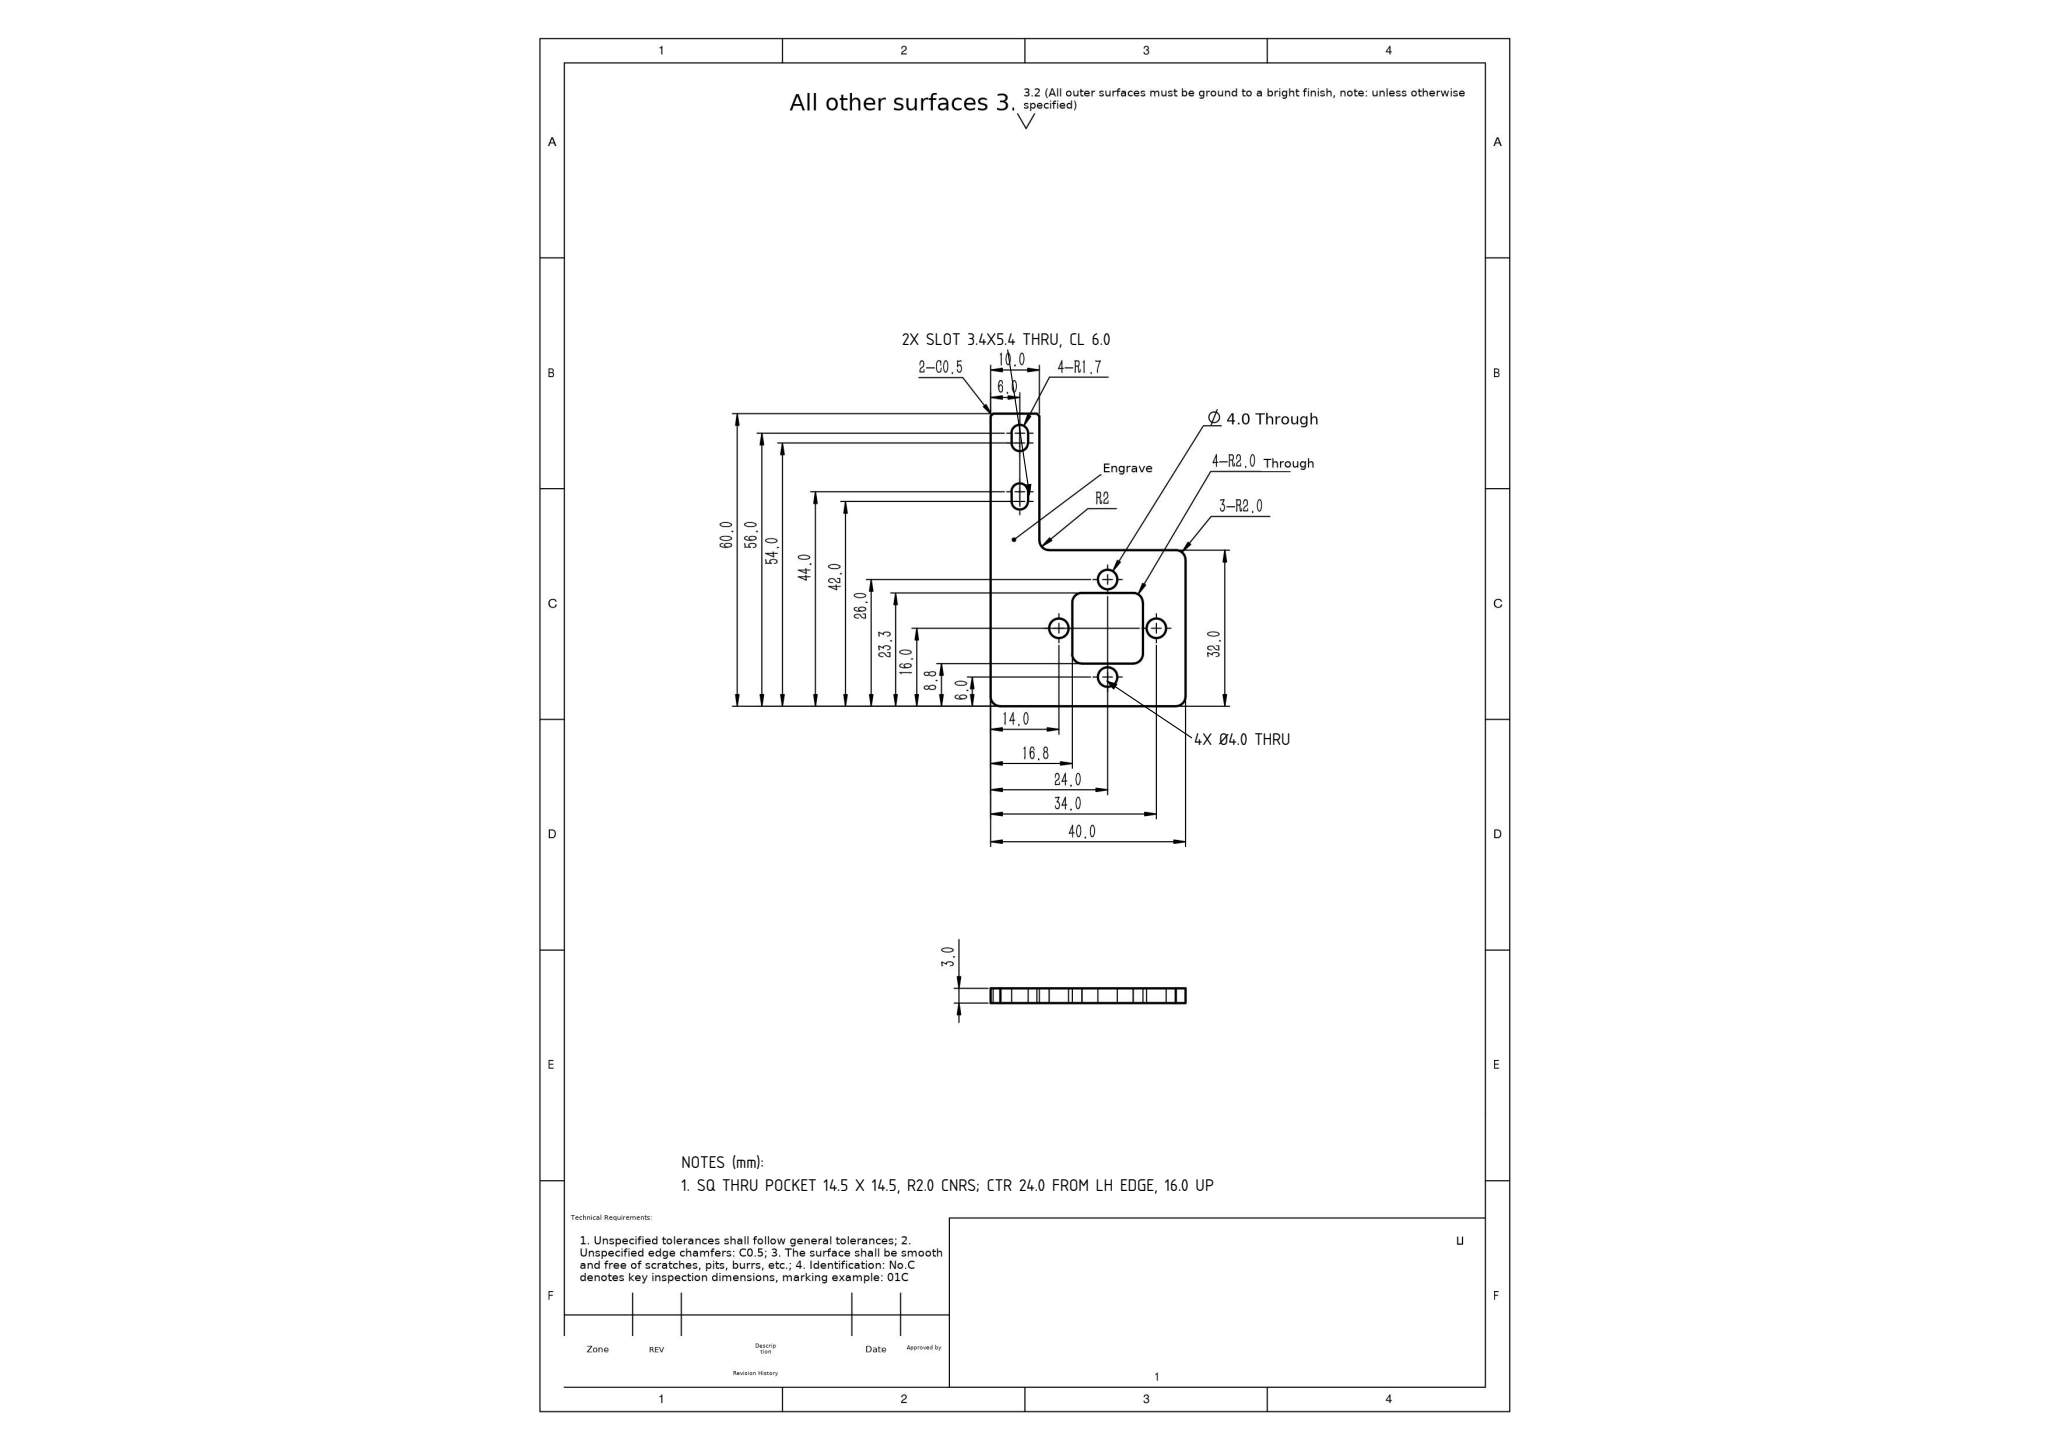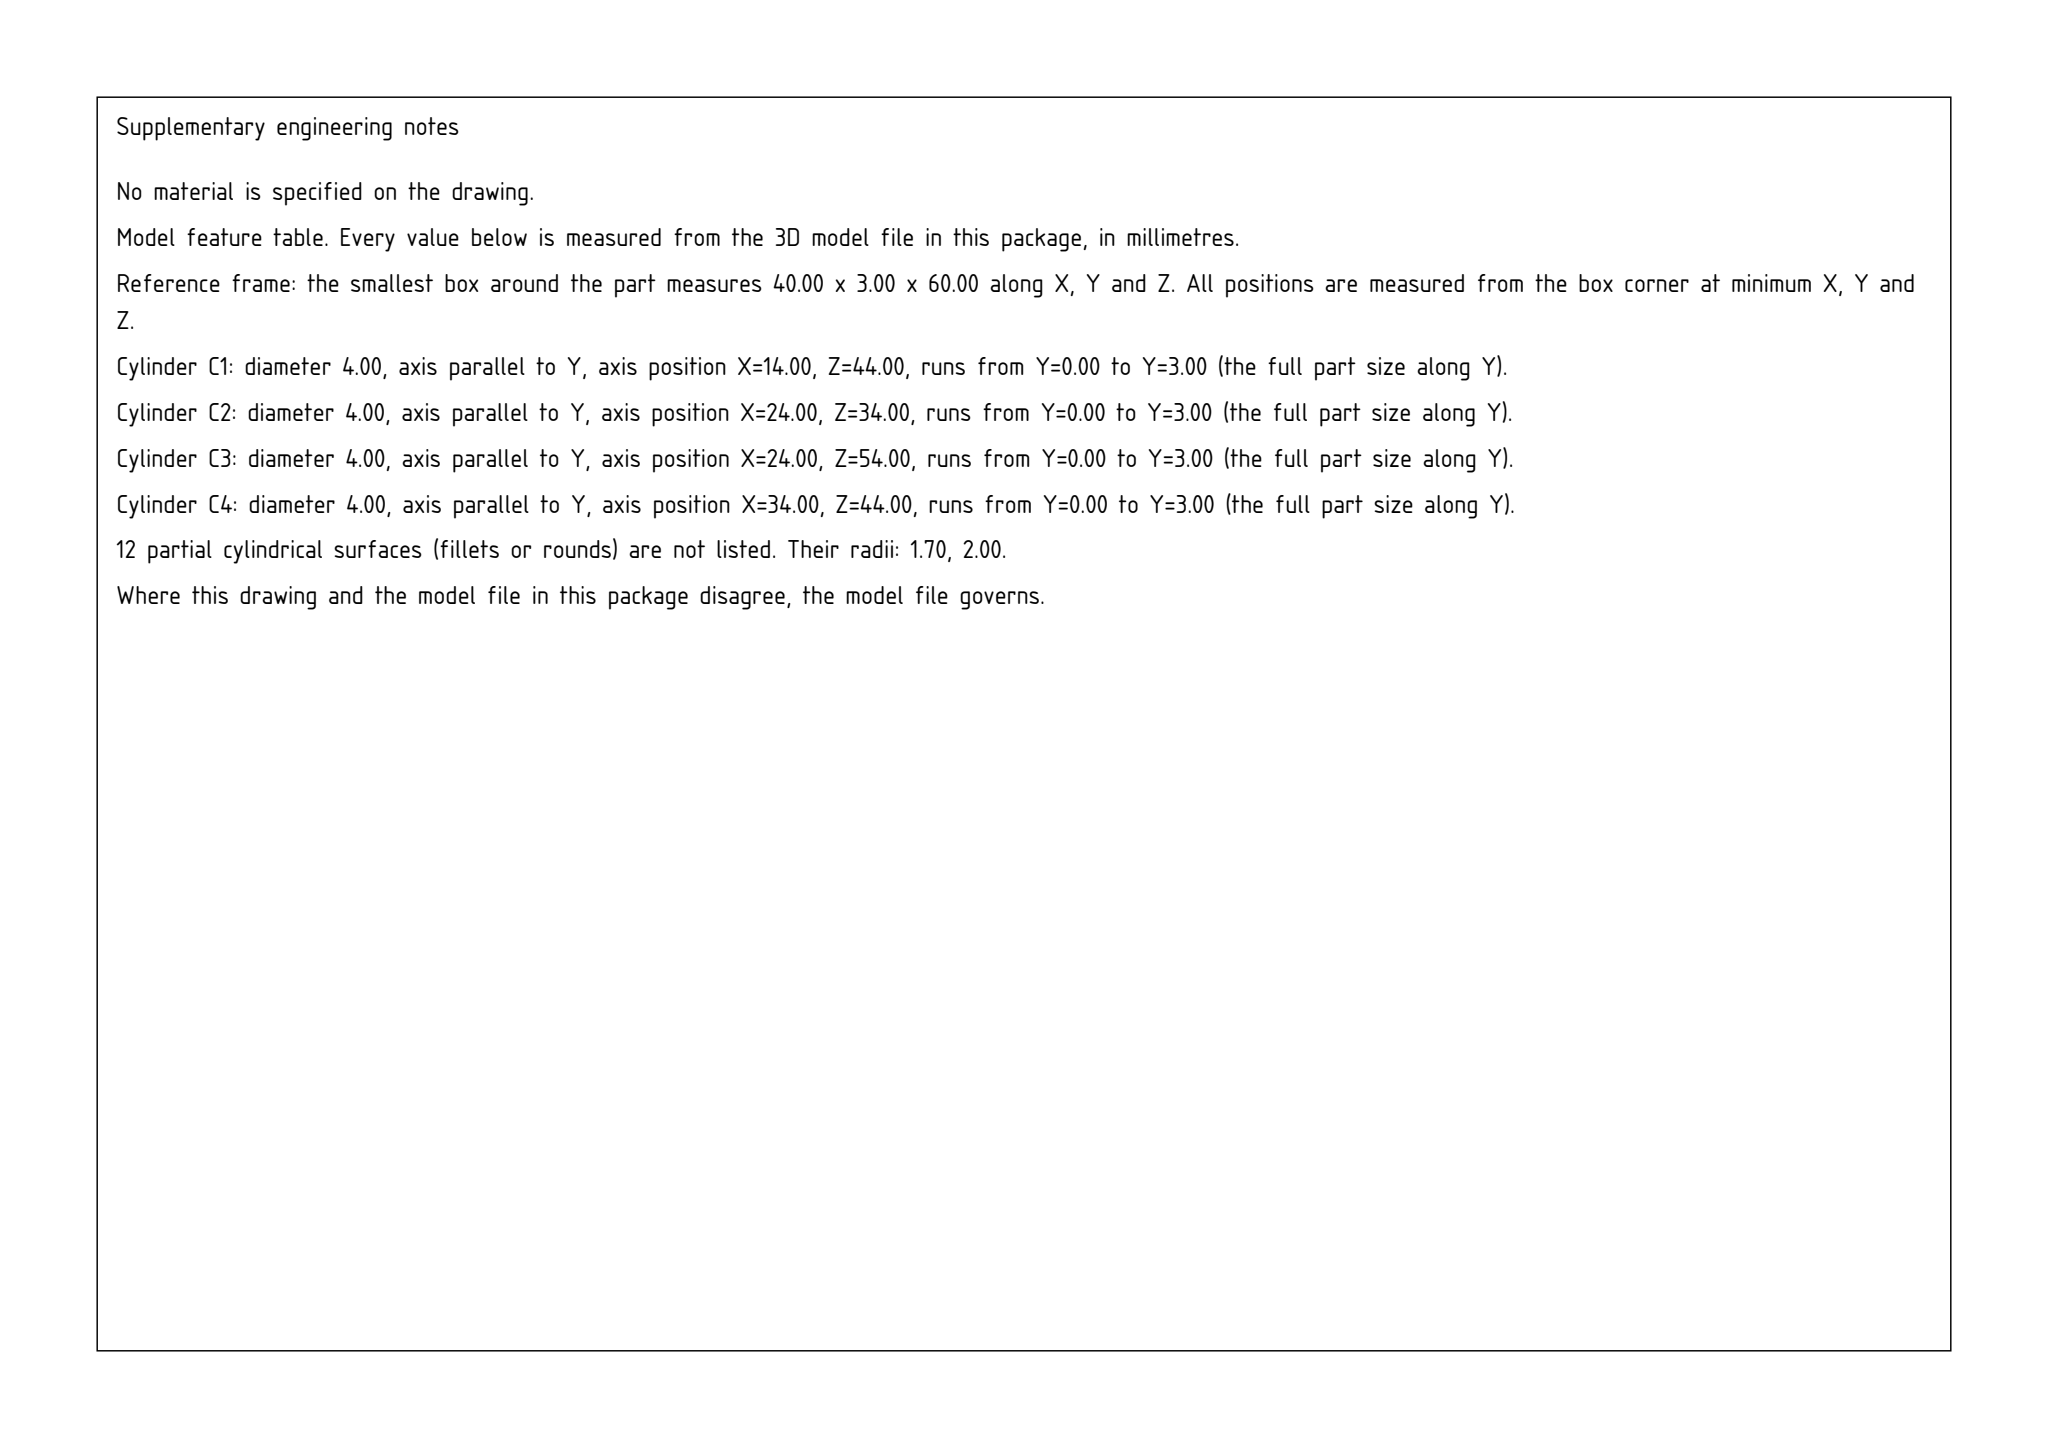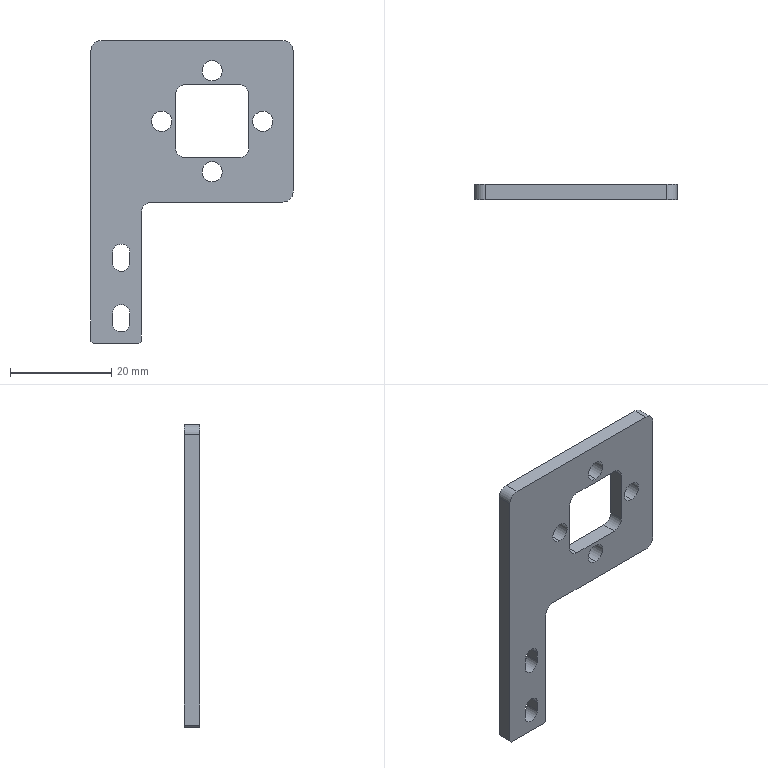Part | SolidWorks | mm | material Alloy Steel | 1 solid | 40 faces | box 40 x 3 x 60 mm | volume 3808 mm3 | cylinder 22 | plane 18 | commonest cylinder face diameters 4 x16 3.4 x6
Drawing notes:
4-R1.7 SLOT: 3.4 W X 5.4 OAL THRU, END CTRS 2.0 APART, CL 6.0 FROM LH EDGE | from the solid: Ø3.4 y-axis cyls at x=6.0, z=4.0/6.0 and z=16.0/18.0; x planes 4.3 & 7.7 => 3.4 W; 2.0 ctr dist + 3.4 = 5.4 OAL
SQ THRU POCKET 14.5 X 14.5, R2.0 CNRS; CTR 24.0 FROM LH EDGE, 16.0 UP | from the solid: x planes 16.75/31.25 and z planes 36.75/51.25 => 14.5 sq; R2.0 corner cyls at (18.75,38.75),(18.75,49.25),(29.25,38.75),(29.25,49.25); ctr x=24.0, z=44.0 => 16.0 from bottom edge
4X Ø4.0 THRU (3.0 thk); hole centers from LH edge / bottom edge: (14.0, 44.0), (24.0, 34.0), (24.0, 54.0), (34.0, 44.0) | from the solid: cylinders dia 4.0, axis y, length 3.0 (full 3.0 thickness) at pos (14.0,44.0), (24.0,34.0), (24.0,54.0), (34.0,44.0)
build123d program:
from build123d import *

# Parameters (mm, degrees)
SKETCH1_R           = 2
SKETCH1_W           = 14.5
SKETCH1_H           = 14.5
BOSS_EXTRUDE1_DEPTH = 3
FILLET1_R           = 2
CUT_EXTRUDE1_DEPTH  = 3
CHAMFER1_SIZE       = 0.5


with BuildPart() as part:
    # Sketch1 → Boss-Extrude1 (new body)
    with BuildSketch(Plane(origin=(0, 0, 0), x_dir=(1, 0, 0), z_dir=(0, 1, 0))):
        Polygon((0, 0), (0, -60), (40, -60), (40, -28), (10, -28), (10, 0), align=None)
        with Locations(Location((24, -34, 0), (0, 0, 270))):
            Circle(SKETCH1_R, mode=Mode.SUBTRACT)
        with Locations(Location((24, -54, 0), (0, 0, 270))):
            Circle(SKETCH1_R, mode=Mode.SUBTRACT)
        with Locations(Location((14, -44, 0), (0, 0, 270))):
            Circle(SKETCH1_R, mode=Mode.SUBTRACT)
        with Locations(Location((34, -44, 0), (0, 0, 270))):
            Circle(SKETCH1_R, mode=Mode.SUBTRACT)
        with Locations((24, -44)):
            Rectangle(SKETCH1_W, SKETCH1_H, mode=Mode.SUBTRACT)
    extrude(amount=BOSS_EXTRUDE1_DEPTH)

    # Fillet1
    fillet1_edges = [part.edges().sort_by_distance(p)[0] for p in [
        (10, 1.5, 28),
        (40, 1.5, 28),
        (40, 1.5, 60),
        (0, 1.5, 60),
        (31.25, 1.5, 51.25),
        (31.25, 1.5, 36.75),
        (16.75, 1.5, 36.75),
        (16.75, 1.5, 51.25),
    ]]
    fillet(fillet1_edges, radius=FILLET1_R)

    # Sketch2 → Cut-Extrude1 (cut)
    with BuildSketch(Plane(origin=(0, 3, 0), x_dir=(1, 0, 0), z_dir=(0, 1, 0))):
        with BuildLine():
            Line((7.7, -4), (7.7, -6))
            ThreePointArc((7.7, -6), (6, -7.7), (4.3, -6))
            Line((4.3, -6), (4.3, -4))
            ThreePointArc((4.3, -4), (6, -2.3), (7.7, -4))
        make_face()
        with BuildLine():
            Line((7.7, -16), (7.7, -18))
            ThreePointArc((7.7, -18), (6, -19.7), (4.3, -18))
            Line((4.3, -18), (4.3, -16))
            ThreePointArc((4.3, -16), (6, -14.3), (7.7, -16))
        make_face()
    extrude(amount=-CUT_EXTRUDE1_DEPTH, mode=Mode.SUBTRACT)

    # Chamfer1
    chamfer1_edges = [part.edges().sort_by_distance(p)[0] for p in [
        (10, 1.5, 0),
        (0, 1.5, 0),
    ]]
    chamfer(chamfer1_edges, length=CHAMFER1_SIZE)


solid = part.part